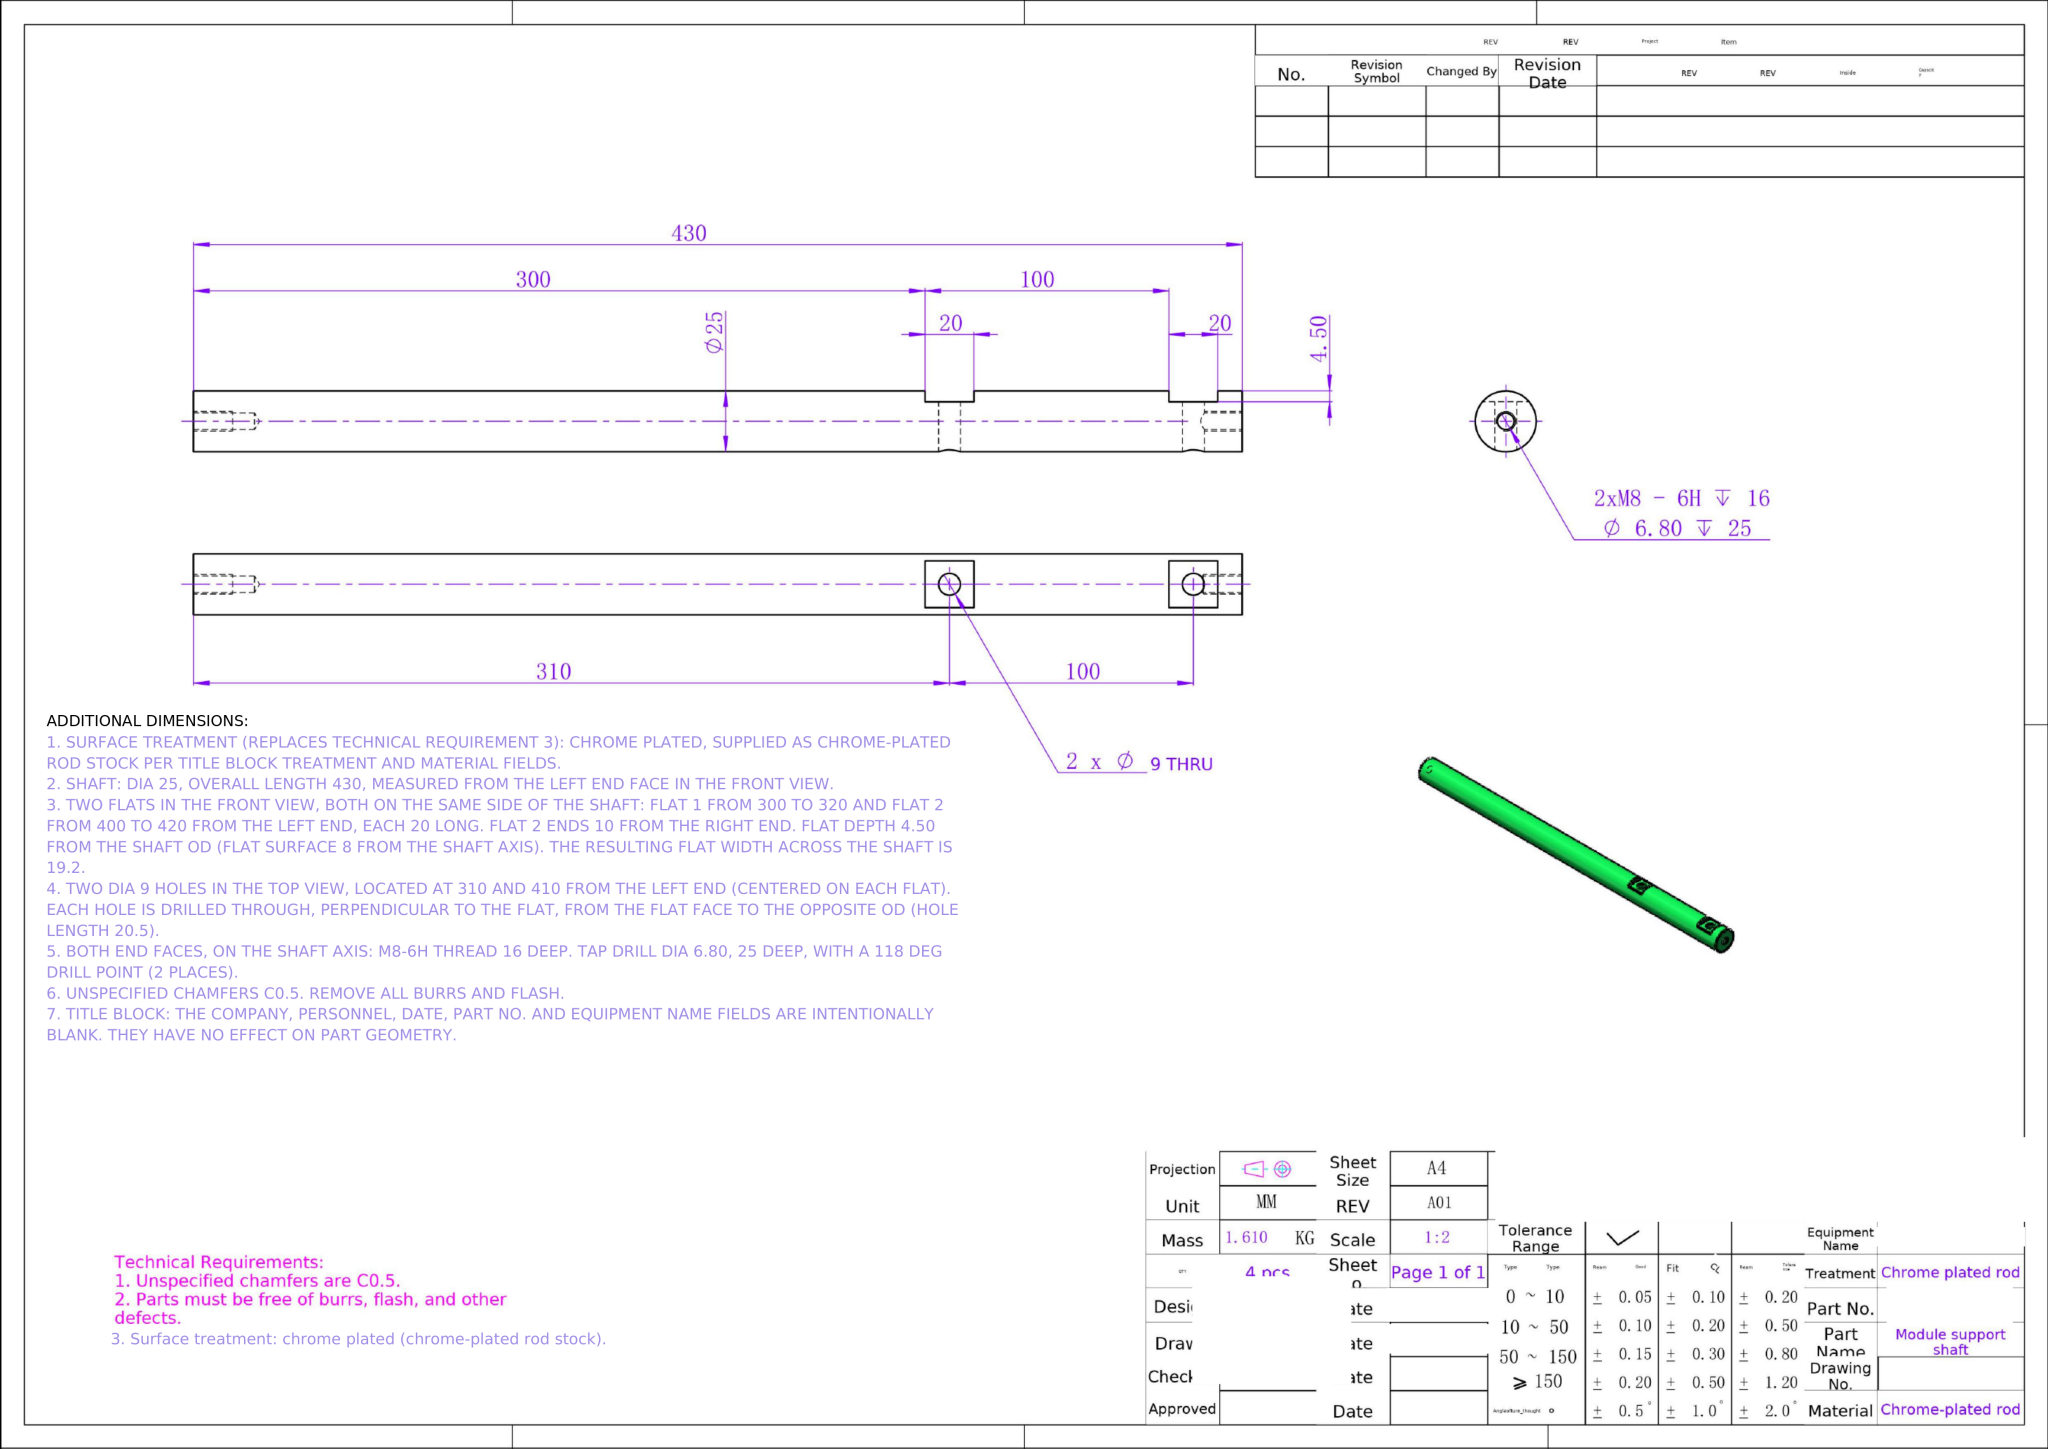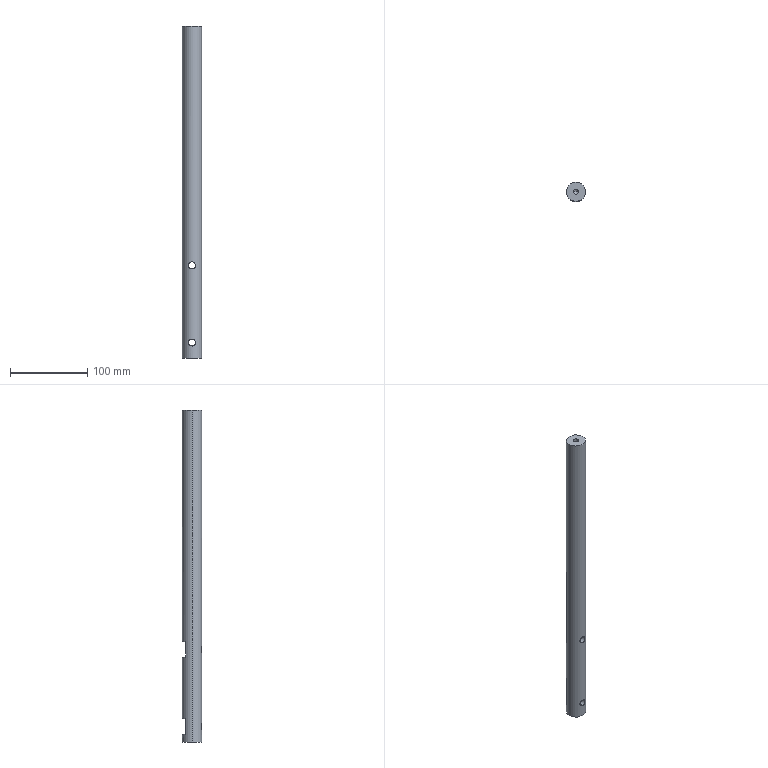Part | NX | mm | Dual-Bore Cylindrical Support Rod | 1 solid | 20 faces | box 25 x 25 x 430 mm | volume 204582 mm3 | cylinder 10 | plane 8 | cone 2 | commonest cylinder face diameters 6.8 x4 9 x4 25 x2
STEP:
#1=CARTESIAN_POINT('',(43.4,-10.,-412.948));
#2=VERTEX_POINT('',#1);
#3=CARTESIAN_POINT('',(40.,-13.4,-414.5));
#4=VERTEX_POINT('',#3);
#5=CARTESIAN_POINT('',(43.4,-10.,-412.948));
#6=CARTESIAN_POINT('',(43.4,-10.117,-412.948));
#7=CARTESIAN_POINT('',(43.394,-10.235,-412.955));
#8=CARTESIAN_POINT('',(43.37,-10.467,-412.982));
#9=CARTESIAN_POINT('',(43.352,-10.581,-413.003));
#10=CARTESIAN_POINT('',(43.282,-10.916,-413.079));
#11=CARTESIAN_POINT('',(43.214,-11.132,-413.152));
#12=CARTESIAN_POINT('',(42.958,-11.733,-413.4));
#13=CARTESIAN_POINT('',(42.716,-12.089,-413.605));
#14=CARTESIAN_POINT('',(42.267,-12.542,-413.891));
#15=CARTESIAN_POINT('',(42.101,-12.682,-413.984));
#16=CARTESIAN_POINT('',(41.742,-12.928,-414.154));
#17=CARTESIAN_POINT('',(41.549,-13.035,-414.23));
#18=CARTESIAN_POINT('',(41.137,-13.212,-414.359));
#19=CARTESIAN_POINT('',(40.916,-13.282,-414.412));
#20=CARTESIAN_POINT('',(40.468,-13.375,-414.481));
#21=CARTESIAN_POINT('',(40.235,-13.4,-414.5));
#22=CARTESIAN_POINT('',(40.,-13.4,-414.5));
#23=B_SPLINE_CURVE_WITH_KNOTS('',3,(#5,#6,#7,#8,#9,#10,#11,#12,#13,#14,#15,#16,#17,#18,#19,#20,#21,#22),.UNSPECIFIED.,.F.,.F.,(4,2,2,2,2,2,2,2,4),(0.01113,0.01148,0.01183,0.01252,0.01391,0.01461,0.0153,0.016,0.01669),.UNSPECIFIED.);
#24=EDGE_CURVE('',#2,#4,#23,.T.);
#25=ORIENTED_EDGE('',*,*,#24,.F.);
#26=CARTESIAN_POINT('',(43.4,-10.,-430.));
#27=VERTEX_POINT('',#26);
#28=CARTESIAN_POINT('',(43.4,-10.,-430.));
#29=DIRECTION('',(0.,0.,-1.));
#30=VECTOR('',#29,1000.);
#31=LINE('',#28,#30);
#32=EDGE_CURVE('',#2,#27,#31,.T.);
#33=ORIENTED_EDGE('',*,*,#32,.T.);
#34=CARTESIAN_POINT('',(36.6,-10.,-430.));
#35=VERTEX_POINT('',#34);
#36=CARTESIAN_POINT('',(40.,-10.,-430.));
#37=DIRECTION('',(0.,0.,-1.));
#38=DIRECTION('',(-1.,0.,0.));
#39=AXIS2_PLACEMENT_3D('',#36,#37,#38);
#40=CIRCLE('',#39,3.4);
#41=EDGE_CURVE('',#27,#35,#40,.T.);
#42=ORIENTED_EDGE('',*,*,#41,.T.);
#43=CARTESIAN_POINT('',(36.6,-10.,-412.948));
#44=VERTEX_POINT('',#43);
#45=CARTESIAN_POINT('',(36.6,-10.,-430.));
#46=DIRECTION('',(0.,0.,-1.));
#47=VECTOR('',#46,1000.);
#48=LINE('',#45,#47);
#49=EDGE_CURVE('',#44,#35,#48,.T.);
#50=ORIENTED_EDGE('',*,*,#49,.F.);
#51=CARTESIAN_POINT('',(40.,-13.4,-414.5));
#52=CARTESIAN_POINT('',(39.765,-13.4,-414.5));
#53=CARTESIAN_POINT('',(39.535,-13.376,-414.482));
#54=CARTESIAN_POINT('',(39.083,-13.282,-414.411));
#55=CARTESIAN_POINT('',(38.862,-13.212,-414.359));
#56=CARTESIAN_POINT('',(38.451,-13.035,-414.231));
#57=CARTESIAN_POINT('',(38.255,-12.926,-414.153));
#58=CARTESIAN_POINT('',(37.897,-12.68,-413.983));
#59=CARTESIAN_POINT('',(37.733,-12.543,-413.891));
#60=CARTESIAN_POINT('',(37.281,-12.086,-413.604));
#61=CARTESIAN_POINT('',(37.044,-11.736,-413.401));
#62=CARTESIAN_POINT('',(36.785,-11.129,-413.151));
#63=CARTESIAN_POINT('',(36.718,-10.918,-413.08));
#64=CARTESIAN_POINT('',(36.625,-10.47,-412.977));
#65=CARTESIAN_POINT('',(36.6,-10.236,-412.948));
#66=CARTESIAN_POINT('',(36.6,-10.,-412.948));
#67=B_SPLINE_CURVE_WITH_KNOTS('',3,(#51,#52,#53,#54,#55,#56,#57,#58,#59,#60,#61,#62,#63,#64,#65,#66),.UNSPECIFIED.,.F.,.F.,(4,2,2,2,2,2,2,4),(0.01669,0.01739,0.01808,0.01878,0.01947,0.02086,0.02155,0.02225),.UNSPECIFIED.);
#68=EDGE_CURVE('',#4,#44,#67,.T.);
#69=ORIENTED_EDGE('',*,*,#68,.F.);
#70=EDGE_LOOP('',(#25,#33,#42,#50,#69));
#71=FACE_OUTER_BOUND('',#70,.T.);
#72=CARTESIAN_POINT('',(40.,-10.,-430.));
#73=DIRECTION('',(0.,0.,-1.));
#74=DIRECTION('',(-1.,0.,0.));
#75=AXIS2_PLACEMENT_3D('',#72,#73,#74);
#76=CYLINDRICAL_SURFACE('',#75,3.4);
#77=ADVANCED_FACE('',(#71),#76,.F.);
#78=CARTESIAN_POINT('',(36.6,-10.,-25.));
#79=VERTEX_POINT('',#78);
#80=CARTESIAN_POINT('',(43.4,-10.,-25.));
#81=VERTEX_POINT('',#80);
#82=CARTESIAN_POINT('',(40.,-10.,-25.));
#83=DIRECTION('',(0.,0.,1.));
#84=DIRECTION('',(1.,0.,0.));
#85=AXIS2_PLACEMENT_3D('',#82,#83,#84);
#86=CIRCLE('',#85,3.4);
#87=EDGE_CURVE('',#79,#81,#86,.T.);
#88=ORIENTED_EDGE('',*,*,#87,.F.);
#89=CARTESIAN_POINT('',(36.6,-10.,0.));
#90=VERTEX_POINT('',#89);
#91=CARTESIAN_POINT('',(36.6,-10.,0.));
#92=DIRECTION('',(0.,0.,1.));
#93=VECTOR('',#92,1000.);
#94=LINE('',#91,#93);
#95=EDGE_CURVE('',#79,#90,#94,.T.);
#96=ORIENTED_EDGE('',*,*,#95,.T.);
#97=CARTESIAN_POINT('',(43.4,-10.,0.));
#98=VERTEX_POINT('',#97);
#99=CARTESIAN_POINT('',(40.,-10.,0.));
#100=DIRECTION('',(0.,0.,1.));
#101=DIRECTION('',(1.,0.,0.));
#102=AXIS2_PLACEMENT_3D('',#99,#100,#101);
#103=CIRCLE('',#102,3.4);
#104=EDGE_CURVE('',#90,#98,#103,.T.);
#105=ORIENTED_EDGE('',*,*,#104,.T.);
#106=CARTESIAN_POINT('',(43.4,-10.,0.));
#107=DIRECTION('',(0.,0.,1.));
#108=VECTOR('',#107,1000.);
#109=LINE('',#106,#108);
#110=EDGE_CURVE('',#81,#98,#109,.T.);
#111=ORIENTED_EDGE('',*,*,#110,.F.);
#112=EDGE_LOOP('',(#88,#96,#105,#111));
#113=FACE_OUTER_BOUND('',#112,.T.);
#114=CARTESIAN_POINT('',(40.,-10.,0.));
#115=DIRECTION('',(0.,0.,1.));
#116=DIRECTION('',(1.,0.,0.));
#117=AXIS2_PLACEMENT_3D('',#114,#115,#116);
#118=CYLINDRICAL_SURFACE('',#117,3.4);
#119=ADVANCED_FACE('',(#113),#118,.F.);
#120=CARTESIAN_POINT('',(40.,-10.,-27.043));
#121=VERTEX_POINT('',#120);
#122=CARTESIAN_POINT('',(43.4,-10.,-25.));
#123=DIRECTION('',(0.8572,0.,0.515));
#124=VECTOR('',#123,1000.);
#125=LINE('',#122,#124);
#126=EDGE_CURVE('',#121,#81,#125,.T.);
#127=ORIENTED_EDGE('',*,*,#126,.F.);
#128=CARTESIAN_POINT('',(36.6,-10.,-25.));
#129=DIRECTION('',(-0.8572,0.,0.515));
#130=VECTOR('',#129,1000.);
#131=LINE('',#128,#130);
#132=EDGE_CURVE('',#121,#79,#131,.T.);
#133=ORIENTED_EDGE('',*,*,#132,.T.);
#134=ORIENTED_EDGE('',*,*,#87,.T.);
#135=EDGE_LOOP('',(#127,#133,#134));
#136=FACE_OUTER_BOUND('',#135,.T.);
#137=CARTESIAN_POINT('',(40.,-10.,-25.));
#138=DIRECTION('',(0.,0.,1.));
#139=DIRECTION('',(1.,0.,0.));
#140=AXIS2_PLACEMENT_3D('',#137,#138,#139);
#141=CONICAL_SURFACE('',#140,3.4,1.03);
#142=ADVANCED_FACE('',(#136),#141,.F.);
#143=CARTESIAN_POINT('',(40.,-22.5,-405.5));
#144=VERTEX_POINT('',#143);
#145=CARTESIAN_POINT('',(40.,-22.5,-414.5));
#146=VERTEX_POINT('',#145);
#147=CARTESIAN_POINT('',(40.,-22.5,-405.5));
#148=CARTESIAN_POINT('',(39.7,-22.5,-405.5));
#149=CARTESIAN_POINT('',(39.405,-22.489,-405.53));
#150=CARTESIAN_POINT('',(38.827,-22.448,-405.646));
#151=CARTESIAN_POINT('',(38.539,-22.417,-405.733));
#152=CARTESIAN_POINT('',(37.995,-22.341,-405.96));
#153=CARTESIAN_POINT('',(37.738,-22.296,-406.099));
#154=CARTESIAN_POINT('',(37.251,-22.196,-406.426));
#155=CARTESIAN_POINT('',(37.022,-22.142,-406.614));
#156=CARTESIAN_POINT('',(36.611,-22.034,-407.025));
#157=CARTESIAN_POINT('',(36.425,-21.979,-407.251));
#158=CARTESIAN_POINT('',(36.097,-21.876,-407.741));
#159=CARTESIAN_POINT('',(35.959,-21.829,-407.999));
#160=CARTESIAN_POINT('',(35.79,-21.77,-408.404));
#161=CARTESIAN_POINT('',(35.74,-21.752,-408.542));
#162=CARTESIAN_POINT('',(35.653,-21.72,-408.825));
#163=CARTESIAN_POINT('',(35.617,-21.706,-408.971));
#164=CARTESIAN_POINT('',(35.529,-21.673,-409.408));
#165=CARTESIAN_POINT('',(35.5,-21.662,-409.701));
#166=CARTESIAN_POINT('',(35.5,-21.662,-410.294));
#167=CARTESIAN_POINT('',(35.53,-21.673,-410.595));
#168=CARTESIAN_POINT('',(35.646,-21.717,-411.174));
#169=CARTESIAN_POINT('',(35.732,-21.749,-411.456));
#170=CARTESIAN_POINT('',(35.96,-21.83,-412.004));
#171=CARTESIAN_POINT('',(36.099,-21.877,-412.263));
#172=CARTESIAN_POINT('',(36.424,-21.979,-412.748));
#173=CARTESIAN_POINT('',(36.613,-22.034,-412.977));
#174=CARTESIAN_POINT('',(37.026,-22.143,-413.39));
#175=CARTESIAN_POINT('',(37.251,-22.196,-413.574));
#176=CARTESIAN_POINT('',(37.737,-22.296,-413.9));
#177=CARTESIAN_POINT('',(38.,-22.342,-414.042));
#178=CARTESIAN_POINT('',(38.541,-22.418,-414.267));
#179=CARTESIAN_POINT('',(38.823,-22.448,-414.353));
#180=CARTESIAN_POINT('',(39.407,-22.489,-414.471));
#181=CARTESIAN_POINT('',(39.704,-22.5,-414.5));
#182=CARTESIAN_POINT('',(40.,-22.5,-414.5));
#183=B_SPLINE_CURVE_WITH_KNOTS('',3,(#147,#148,#149,#150,#151,#152,#153,#154,#155,#156,#157,#158,#159,#160,#161,#162,#163,#164,#165,#166,#167,#168,#169,#170,#171,#172,#173,#174,#175,#176,#177,#178,#179,#180,#181,#182),.UNSPECIFIED.,.F.,.F.,(4,2,2,2,2,2,2,2,2,2,2,2,2,2,2,2,2,4),(0.,0.0008868,0.001774,0.00266,0.003547,0.004434,0.005321,0.005764,0.006208,0.007095,0.007981,0.008868,0.009755,0.01064,0.01153,0.01242,0.0133,0.01419),.UNSPECIFIED.);
#184=EDGE_CURVE('',#144,#146,#183,.T.);
#185=ORIENTED_EDGE('',*,*,#184,.T.);
#186=CARTESIAN_POINT('',(40.,-2.,-414.5));
#187=DIRECTION('',(0.,1.,0.));
#188=VECTOR('',#187,1000.);
#189=LINE('',#186,#188);
#190=EDGE_CURVE('',#146,#4,#189,.T.);
#191=ORIENTED_EDGE('',*,*,#190,.T.);
#192=ORIENTED_EDGE('',*,*,#68,.T.);
#193=CARTESIAN_POINT('',(40.,-6.6,-414.5));
#194=VERTEX_POINT('',#193);
#195=CARTESIAN_POINT('',(36.6,-10.,-412.948));
#196=CARTESIAN_POINT('',(36.6,-9.763,-412.948));
#197=CARTESIAN_POINT('',(36.624,-9.534,-412.977));
#198=CARTESIAN_POINT('',(36.717,-9.088,-413.078));
#199=CARTESIAN_POINT('',(36.785,-8.871,-413.151));
#200=CARTESIAN_POINT('',(37.041,-8.27,-413.398));
#201=CARTESIAN_POINT('',(37.282,-7.913,-413.604));
#202=CARTESIAN_POINT('',(37.731,-7.459,-413.89));
#203=CARTESIAN_POINT('',(37.898,-7.319,-413.984));
#204=CARTESIAN_POINT('',(38.257,-7.073,-414.154));
#205=CARTESIAN_POINT('',(38.449,-6.966,-414.23));
#206=CARTESIAN_POINT('',(38.863,-6.788,-414.359));
#207=CARTESIAN_POINT('',(39.083,-6.718,-414.411));
#208=CARTESIAN_POINT('',(39.532,-6.625,-414.481));
#209=CARTESIAN_POINT('',(39.765,-6.6,-414.5));
#210=CARTESIAN_POINT('',(40.,-6.6,-414.5));
#211=B_SPLINE_CURVE_WITH_KNOTS('',3,(#195,#196,#197,#198,#199,#200,#201,#202,#203,#204,#205,#206,#207,#208,#209,#210),.UNSPECIFIED.,.F.,.F.,(4,2,2,2,2,2,2,4),(0.,0.0006966,0.001393,0.002786,0.003483,0.004179,0.004876,0.005573),.UNSPECIFIED.);
#212=EDGE_CURVE('',#44,#194,#211,.T.);
#213=ORIENTED_EDGE('',*,*,#212,.T.);
#214=CARTESIAN_POINT('',(40.,-2.,-414.5));
#215=VERTEX_POINT('',#214);
#216=CARTESIAN_POINT('',(40.,-2.,-414.5));
#217=DIRECTION('',(0.,1.,0.));
#218=VECTOR('',#217,1000.);
#219=LINE('',#216,#218);
#220=EDGE_CURVE('',#194,#215,#219,.T.);
#221=ORIENTED_EDGE('',*,*,#220,.T.);
#222=CARTESIAN_POINT('',(40.,-2.,-405.5));
#223=VERTEX_POINT('',#222);
#224=CARTESIAN_POINT('',(40.,-2.,-410.));
#225=DIRECTION('',(0.,1.,0.));
#226=DIRECTION('',(0.,0.,1.));
#227=AXIS2_PLACEMENT_3D('',#224,#225,#226);
#228=CIRCLE('',#227,4.5);
#229=EDGE_CURVE('',#215,#223,#228,.T.);
#230=ORIENTED_EDGE('',*,*,#229,.T.);
#231=CARTESIAN_POINT('',(40.,-2.,-405.5));
#232=DIRECTION('',(0.,1.,0.));
#233=VECTOR('',#232,1000.);
#234=LINE('',#231,#233);
#235=EDGE_CURVE('',#144,#223,#234,.T.);
#236=ORIENTED_EDGE('',*,*,#235,.F.);
#237=EDGE_LOOP('',(#185,#191,#192,#213,#221,#230,#236));
#238=FACE_OUTER_BOUND('',#237,.T.);
#239=CARTESIAN_POINT('',(40.,-2.,-410.));
#240=DIRECTION('',(0.,1.,0.));
#241=DIRECTION('',(0.,0.,1.));
#242=AXIS2_PLACEMENT_3D('',#239,#240,#241);
#243=CYLINDRICAL_SURFACE('',#242,4.5);
#244=ADVANCED_FACE('',(#238),#243,.F.);
#245=CARTESIAN_POINT('',(40.,-22.5,-305.5));
#246=VERTEX_POINT('',#245);
#247=CARTESIAN_POINT('',(40.,-22.5,-314.5));
#248=VERTEX_POINT('',#247);
#249=CARTESIAN_POINT('',(40.,-22.5,-305.5));
#250=CARTESIAN_POINT('',(39.7,-22.5,-305.5));
#251=CARTESIAN_POINT('',(39.405,-22.489,-305.53));
#252=CARTESIAN_POINT('',(38.827,-22.448,-305.646));
#253=CARTESIAN_POINT('',(38.539,-22.417,-305.733));
#254=CARTESIAN_POINT('',(37.995,-22.341,-305.96));
#255=CARTESIAN_POINT('',(37.738,-22.296,-306.099));
#256=CARTESIAN_POINT('',(37.251,-22.196,-306.426));
#257=CARTESIAN_POINT('',(37.022,-22.142,-306.614));
#258=CARTESIAN_POINT('',(36.611,-22.034,-307.025));
#259=CARTESIAN_POINT('',(36.425,-21.979,-307.251));
#260=CARTESIAN_POINT('',(36.097,-21.876,-307.741));
#261=CARTESIAN_POINT('',(35.959,-21.829,-307.999));
#262=CARTESIAN_POINT('',(35.79,-21.77,-308.404));
#263=CARTESIAN_POINT('',(35.74,-21.752,-308.542));
#264=CARTESIAN_POINT('',(35.653,-21.72,-308.825));
#265=CARTESIAN_POINT('',(35.617,-21.706,-308.971));
#266=CARTESIAN_POINT('',(35.529,-21.673,-309.408));
#267=CARTESIAN_POINT('',(35.5,-21.662,-309.701));
#268=CARTESIAN_POINT('',(35.5,-21.662,-310.294));
#269=CARTESIAN_POINT('',(35.53,-21.673,-310.595));
#270=CARTESIAN_POINT('',(35.646,-21.717,-311.174));
#271=CARTESIAN_POINT('',(35.732,-21.749,-311.456));
#272=CARTESIAN_POINT('',(35.96,-21.83,-312.004));
#273=CARTESIAN_POINT('',(36.099,-21.877,-312.263));
#274=CARTESIAN_POINT('',(36.424,-21.979,-312.748));
#275=CARTESIAN_POINT('',(36.613,-22.034,-312.977));
#276=CARTESIAN_POINT('',(37.026,-22.143,-313.39));
#277=CARTESIAN_POINT('',(37.251,-22.196,-313.574));
#278=CARTESIAN_POINT('',(37.737,-22.296,-313.9));
#279=CARTESIAN_POINT('',(38.,-22.342,-314.042));
#280=CARTESIAN_POINT('',(38.541,-22.418,-314.267));
#281=CARTESIAN_POINT('',(38.823,-22.448,-314.353));
#282=CARTESIAN_POINT('',(39.407,-22.489,-314.471));
#283=CARTESIAN_POINT('',(39.704,-22.5,-314.5));
#284=CARTESIAN_POINT('',(40.,-22.5,-314.5));
#285=B_SPLINE_CURVE_WITH_KNOTS('',3,(#249,#250,#251,#252,#253,#254,#255,#256,#257,#258,#259,#260,#261,#262,#263,#264,#265,#266,#267,#268,#269,#270,#271,#272,#273,#274,#275,#276,#277,#278,#279,#280,#281,#282,#283,#284),.UNSPECIFIED.,.F.,.F.,(4,2,2,2,2,2,2,2,2,2,2,2,2,2,2,2,2,4),(0.,0.0008868,0.001774,0.00266,0.003547,0.004434,0.005321,0.005764,0.006208,0.007095,0.007981,0.008868,0.009755,0.01064,0.01153,0.01242,0.0133,0.01419),.UNSPECIFIED.);
#286=EDGE_CURVE('',#246,#248,#285,.T.);
#287=ORIENTED_EDGE('',*,*,#286,.T.);
#288=CARTESIAN_POINT('',(40.,-2.,-314.5));
#289=VERTEX_POINT('',#288);
#290=CARTESIAN_POINT('',(40.,-2.,-314.5));
#291=DIRECTION('',(0.,1.,0.));
#292=VECTOR('',#291,1000.);
#293=LINE('',#290,#292);
#294=EDGE_CURVE('',#248,#289,#293,.T.);
#295=ORIENTED_EDGE('',*,*,#294,.T.);
#296=CARTESIAN_POINT('',(40.,-2.,-305.5));
#297=VERTEX_POINT('',#296);
#298=CARTESIAN_POINT('',(40.,-2.,-310.));
#299=DIRECTION('',(0.,1.,0.));
#300=DIRECTION('',(0.,0.,1.));
#301=AXIS2_PLACEMENT_3D('',#298,#299,#300);
#302=CIRCLE('',#301,4.5);
#303=EDGE_CURVE('',#289,#297,#302,.T.);
#304=ORIENTED_EDGE('',*,*,#303,.T.);
#305=CARTESIAN_POINT('',(40.,-2.,-305.5));
#306=DIRECTION('',(0.,1.,0.));
#307=VECTOR('',#306,1000.);
#308=LINE('',#305,#307);
#309=EDGE_CURVE('',#246,#297,#308,.T.);
#310=ORIENTED_EDGE('',*,*,#309,.F.);
#311=EDGE_LOOP('',(#287,#295,#304,#310));
#312=FACE_OUTER_BOUND('',#311,.T.);
#313=CARTESIAN_POINT('',(40.,-2.,-310.));
#314=DIRECTION('',(0.,1.,0.));
#315=DIRECTION('',(0.,0.,1.));
#316=AXIS2_PLACEMENT_3D('',#313,#314,#315);
#317=CYLINDRICAL_SURFACE('',#316,4.5);
#318=ADVANCED_FACE('',(#312),#317,.F.);
#319=CARTESIAN_POINT('',(30.395,-2.,-400.));
#320=VERTEX_POINT('',#319);
#321=CARTESIAN_POINT('',(49.605,-2.,-400.));
#322=VERTEX_POINT('',#321);
#323=CARTESIAN_POINT('',(40.,-10.,-400.));
#324=DIRECTION('',(0.,0.,-1.));
#325=DIRECTION('',(1.,0.,0.));
#326=AXIS2_PLACEMENT_3D('',#323,#324,#325);
#327=CIRCLE('',#326,12.5);
#328=EDGE_CURVE('',#320,#322,#327,.T.);
#329=ORIENTED_EDGE('',*,*,#328,.F.);
#330=CARTESIAN_POINT('',(30.395,-2.,-420.));
#331=VERTEX_POINT('',#330);
#332=CARTESIAN_POINT('',(30.395,-2.,-430.));
#333=DIRECTION('',(0.,0.,1.));
#334=VECTOR('',#333,1000.);
#335=LINE('',#332,#334);
#336=EDGE_CURVE('',#331,#320,#335,.T.);
#337=ORIENTED_EDGE('',*,*,#336,.F.);
#338=CARTESIAN_POINT('',(49.605,-2.,-420.));
#339=VERTEX_POINT('',#338);
#340=CARTESIAN_POINT('',(40.,-10.,-420.));
#341=DIRECTION('',(0.,0.,-1.));
#342=DIRECTION('',(1.,0.,0.));
#343=AXIS2_PLACEMENT_3D('',#340,#341,#342);
#344=CIRCLE('',#343,12.5);
#345=EDGE_CURVE('',#331,#339,#344,.T.);
#346=ORIENTED_EDGE('',*,*,#345,.T.);
#347=CARTESIAN_POINT('',(49.605,-2.,-430.));
#348=DIRECTION('',(0.,0.,-1.));
#349=VECTOR('',#348,1000.);
#350=LINE('',#347,#349);
#351=EDGE_CURVE('',#322,#339,#350,.T.);
#352=ORIENTED_EDGE('',*,*,#351,.F.);
#353=EDGE_LOOP('',(#329,#337,#346,#352));
#354=FACE_BOUND('',#353,.T.);
#355=CARTESIAN_POINT('',(30.395,-2.,-300.));
#356=VERTEX_POINT('',#355);
#357=CARTESIAN_POINT('',(49.605,-2.,-300.));
#358=VERTEX_POINT('',#357);
#359=CARTESIAN_POINT('',(40.,-10.,-300.));
#360=DIRECTION('',(0.,0.,-1.));
#361=DIRECTION('',(1.,0.,0.));
#362=AXIS2_PLACEMENT_3D('',#359,#360,#361);
#363=CIRCLE('',#362,12.5);
#364=EDGE_CURVE('',#356,#358,#363,.T.);
#365=ORIENTED_EDGE('',*,*,#364,.F.);
#366=CARTESIAN_POINT('',(30.395,-2.,-320.));
#367=VERTEX_POINT('',#366);
#368=CARTESIAN_POINT('',(30.395,-2.,-330.));
#369=DIRECTION('',(0.,0.,1.));
#370=VECTOR('',#369,1000.);
#371=LINE('',#368,#370);
#372=EDGE_CURVE('',#367,#356,#371,.T.);
#373=ORIENTED_EDGE('',*,*,#372,.F.);
#374=CARTESIAN_POINT('',(49.605,-2.,-320.));
#375=VERTEX_POINT('',#374);
#376=CARTESIAN_POINT('',(40.,-10.,-320.));
#377=DIRECTION('',(0.,0.,-1.));
#378=DIRECTION('',(1.,0.,0.));
#379=AXIS2_PLACEMENT_3D('',#376,#377,#378);
#380=CIRCLE('',#379,12.5);
#381=EDGE_CURVE('',#367,#375,#380,.T.);
#382=ORIENTED_EDGE('',*,*,#381,.T.);
#383=CARTESIAN_POINT('',(49.605,-2.,-330.));
#384=DIRECTION('',(0.,0.,-1.));
#385=VECTOR('',#384,1000.);
#386=LINE('',#383,#385);
#387=EDGE_CURVE('',#358,#375,#386,.T.);
#388=ORIENTED_EDGE('',*,*,#387,.F.);
#389=EDGE_LOOP('',(#365,#373,#382,#388));
#390=FACE_BOUND('',#389,.T.);
#391=CARTESIAN_POINT('',(52.5,-10.,-430.));
#392=VERTEX_POINT('',#391);
#393=CARTESIAN_POINT('',(27.5,-10.,-430.));
#394=VERTEX_POINT('',#393);
#395=CARTESIAN_POINT('',(40.,-10.,-430.));
#396=DIRECTION('',(0.,0.,1.));
#397=DIRECTION('',(1.,0.,0.));
#398=AXIS2_PLACEMENT_3D('',#395,#396,#397);
#399=CIRCLE('',#398,12.5);
#400=EDGE_CURVE('',#392,#394,#399,.T.);
#401=ORIENTED_EDGE('',*,*,#400,.T.);
#402=CARTESIAN_POINT('',(27.5,-10.,0.));
#403=VERTEX_POINT('',#402);
#404=CARTESIAN_POINT('',(27.5,-10.,-430.));
#405=DIRECTION('',(0.,0.,1.));
#406=VECTOR('',#405,1000.);
#407=LINE('',#404,#406);
#408=EDGE_CURVE('',#394,#403,#407,.T.);
#409=ORIENTED_EDGE('',*,*,#408,.T.);
#410=CARTESIAN_POINT('',(52.5,-10.,0.));
#411=VERTEX_POINT('',#410);
#412=CARTESIAN_POINT('',(40.,-10.,0.));
#413=DIRECTION('',(0.,0.,1.));
#414=DIRECTION('',(1.,0.,0.));
#415=AXIS2_PLACEMENT_3D('',#412,#413,#414);
#416=CIRCLE('',#415,12.5);
#417=EDGE_CURVE('',#411,#403,#416,.T.);
#418=ORIENTED_EDGE('',*,*,#417,.F.);
#419=CARTESIAN_POINT('',(52.5,-10.,-430.));
#420=DIRECTION('',(0.,0.,1.));
#421=VECTOR('',#420,1000.);
#422=LINE('',#419,#421);
#423=EDGE_CURVE('',#392,#411,#422,.T.);
#424=ORIENTED_EDGE('',*,*,#423,.F.);
#425=EDGE_LOOP('',(#401,#409,#418,#424));
#426=FACE_OUTER_BOUND('',#425,.T.);
#427=CARTESIAN_POINT('',(40.,-10.,-430.));
#428=DIRECTION('',(0.,0.,1.));
#429=DIRECTION('',(1.,0.,0.));
#430=AXIS2_PLACEMENT_3D('',#427,#428,#429);
#431=CYLINDRICAL_SURFACE('',#430,12.5);
#432=ADVANCED_FACE('',(#354,#390,#426),#431,.T.);
#433=ORIENTED_EDGE('',*,*,#408,.F.);
#434=CARTESIAN_POINT('',(40.,-10.,-430.));
#435=DIRECTION('',(0.,0.,1.));
#436=DIRECTION('',(1.,0.,0.));
#437=AXIS2_PLACEMENT_3D('',#434,#435,#436);
#438=CIRCLE('',#437,12.5);
#439=EDGE_CURVE('',#394,#392,#438,.T.);
#440=ORIENTED_EDGE('',*,*,#439,.T.);
#441=ORIENTED_EDGE('',*,*,#423,.T.);
#442=CARTESIAN_POINT('',(40.,-10.,0.));
#443=DIRECTION('',(0.,0.,1.));
#444=DIRECTION('',(1.,0.,0.));
#445=AXIS2_PLACEMENT_3D('',#442,#443,#444);
#446=CIRCLE('',#445,12.5);
#447=EDGE_CURVE('',#403,#411,#446,.T.);
#448=ORIENTED_EDGE('',*,*,#447,.F.);
#449=EDGE_LOOP('',(#433,#440,#441,#448));
#450=FACE_OUTER_BOUND('',#449,.T.);
#451=ORIENTED_EDGE('',*,*,#184,.F.);
#452=CARTESIAN_POINT('',(40.,-22.5,-414.5));
#453=CARTESIAN_POINT('',(40.295,-22.5,-414.5));
#454=CARTESIAN_POINT('',(40.594,-22.489,-414.471));
#455=CARTESIAN_POINT('',(41.177,-22.448,-414.353));
#456=CARTESIAN_POINT('',(41.459,-22.418,-414.267));
#457=CARTESIAN_POINT('',(42.002,-22.342,-414.041));
#458=CARTESIAN_POINT('',(42.265,-22.296,-413.899));
#459=CARTESIAN_POINT('',(42.75,-22.196,-413.574));
#460=CARTESIAN_POINT('',(42.976,-22.143,-413.388));
#461=CARTESIAN_POINT('',(43.391,-22.033,-412.972));
#462=CARTESIAN_POINT('',(43.577,-21.978,-412.746));
#463=CARTESIAN_POINT('',(43.901,-21.877,-412.262));
#464=CARTESIAN_POINT('',(44.041,-21.829,-412.001));
#465=CARTESIAN_POINT('',(44.268,-21.749,-411.456));
#466=CARTESIAN_POINT('',(44.354,-21.717,-411.175));
#467=CARTESIAN_POINT('',(44.47,-21.674,-410.596));
#468=CARTESIAN_POINT('',(44.5,-21.662,-410.295));
#469=CARTESIAN_POINT('',(44.5,-21.662,-409.702));
#470=CARTESIAN_POINT('',(44.471,-21.673,-409.408));
#471=CARTESIAN_POINT('',(44.354,-21.717,-408.825));
#472=CARTESIAN_POINT('',(44.266,-21.75,-408.539));
#473=CARTESIAN_POINT('',(44.041,-21.83,-407.998));
#474=CARTESIAN_POINT('',(43.9,-21.877,-407.736));
#475=CARTESIAN_POINT('',(43.573,-21.98,-407.249));
#476=CARTESIAN_POINT('',(43.388,-22.034,-407.024));
#477=CARTESIAN_POINT('',(42.975,-22.143,-406.611));
#478=CARTESIAN_POINT('',(42.746,-22.197,-406.423));
#479=CARTESIAN_POINT('',(42.261,-22.296,-406.098));
#480=CARTESIAN_POINT('',(42.003,-22.342,-405.96));
#481=CARTESIAN_POINT('',(41.594,-22.399,-405.789));
#482=CARTESIAN_POINT('',(41.453,-22.416,-405.739));
#483=CARTESIAN_POINT('',(41.17,-22.446,-405.652));
#484=CARTESIAN_POINT('',(41.027,-22.459,-405.616));
#485=CARTESIAN_POINT('',(40.594,-22.489,-405.53));
#486=CARTESIAN_POINT('',(40.3,-22.5,-405.5));
#487=CARTESIAN_POINT('',(40.,-22.5,-405.5));
#488=B_SPLINE_CURVE_WITH_KNOTS('',3,(#452,#453,#454,#455,#456,#457,#458,#459,#460,#461,#462,#463,#464,#465,#466,#467,#468,#469,#470,#471,#472,#473,#474,#475,#476,#477,#478,#479,#480,#481,#482,#483,#484,#485,#486,#487),.UNSPECIFIED.,.F.,.F.,(4,2,2,2,2,2,2,2,2,2,2,2,2,2,2,2,2,4),(0.01419,0.01508,0.01596,0.01685,0.01774,0.01862,0.01951,0.0204,0.02128,0.02217,0.02306,0.02394,0.02483,0.02572,0.0266,0.02705,0.02749,0.02838),.UNSPECIFIED.);
#489=EDGE_CURVE('',#146,#144,#488,.T.);
#490=ORIENTED_EDGE('',*,*,#489,.F.);
#491=EDGE_LOOP('',(#451,#490));
#492=FACE_BOUND('',#491,.T.);
#493=ORIENTED_EDGE('',*,*,#286,.F.);
#494=CARTESIAN_POINT('',(40.,-22.5,-314.5));
#495=CARTESIAN_POINT('',(40.295,-22.5,-314.5));
#496=CARTESIAN_POINT('',(40.594,-22.489,-314.471));
#497=CARTESIAN_POINT('',(41.177,-22.448,-314.353));
#498=CARTESIAN_POINT('',(41.459,-22.418,-314.267));
#499=CARTESIAN_POINT('',(42.002,-22.342,-314.041));
#500=CARTESIAN_POINT('',(42.265,-22.296,-313.899));
#501=CARTESIAN_POINT('',(42.75,-22.196,-313.574));
#502=CARTESIAN_POINT('',(42.976,-22.143,-313.388));
#503=CARTESIAN_POINT('',(43.391,-22.033,-312.972));
#504=CARTESIAN_POINT('',(43.577,-21.978,-312.746));
#505=CARTESIAN_POINT('',(43.901,-21.877,-312.262));
#506=CARTESIAN_POINT('',(44.041,-21.829,-312.001));
#507=CARTESIAN_POINT('',(44.268,-21.749,-311.456));
#508=CARTESIAN_POINT('',(44.354,-21.717,-311.175));
#509=CARTESIAN_POINT('',(44.47,-21.674,-310.596));
#510=CARTESIAN_POINT('',(44.5,-21.662,-310.295));
#511=CARTESIAN_POINT('',(44.5,-21.662,-309.702));
#512=CARTESIAN_POINT('',(44.471,-21.673,-309.408));
#513=CARTESIAN_POINT('',(44.354,-21.717,-308.825));
#514=CARTESIAN_POINT('',(44.266,-21.75,-308.539));
#515=CARTESIAN_POINT('',(44.041,-21.83,-307.998));
#516=CARTESIAN_POINT('',(43.9,-21.877,-307.736));
#517=CARTESIAN_POINT('',(43.573,-21.98,-307.249));
#518=CARTESIAN_POINT('',(43.388,-22.034,-307.024));
#519=CARTESIAN_POINT('',(42.975,-22.143,-306.611));
#520=CARTESIAN_POINT('',(42.746,-22.197,-306.423));
#521=CARTESIAN_POINT('',(42.261,-22.296,-306.098));
#522=CARTESIAN_POINT('',(42.003,-22.342,-305.96));
#523=CARTESIAN_POINT('',(41.594,-22.399,-305.789));
#524=CARTESIAN_POINT('',(41.453,-22.416,-305.739));
#525=CARTESIAN_POINT('',(41.17,-22.446,-305.652));
#526=CARTESIAN_POINT('',(41.027,-22.459,-305.616));
#527=CARTESIAN_POINT('',(40.594,-22.489,-305.53));
#528=CARTESIAN_POINT('',(40.3,-22.5,-305.5));
#529=CARTESIAN_POINT('',(40.,-22.5,-305.5));
#530=B_SPLINE_CURVE_WITH_KNOTS('',3,(#494,#495,#496,#497,#498,#499,#500,#501,#502,#503,#504,#505,#506,#507,#508,#509,#510,#511,#512,#513,#514,#515,#516,#517,#518,#519,#520,#521,#522,#523,#524,#525,#526,#527,#528,#529),.UNSPECIFIED.,.F.,.F.,(4,2,2,2,2,2,2,2,2,2,2,2,2,2,2,2,2,4),(0.01419,0.01508,0.01596,0.01685,0.01774,0.01862,0.01951,0.0204,0.02128,0.02217,0.02306,0.02394,0.02483,0.02572,0.0266,0.02705,0.02749,0.02838),.UNSPECIFIED.);
#531=EDGE_CURVE('',#248,#246,#530,.T.);
#532=ORIENTED_EDGE('',*,*,#531,.F.);
#533=EDGE_LOOP('',(#493,#532));
#534=FACE_BOUND('',#533,.T.);
#535=CARTESIAN_POINT('',(40.,-10.,-430.));
#536=DIRECTION('',(0.,0.,1.));
#537=DIRECTION('',(1.,0.,0.));
#538=AXIS2_PLACEMENT_3D('',#535,#536,#537);
#539=CYLINDRICAL_SURFACE('',#538,12.5);
#540=ADVANCED_FACE('',(#450,#492,#534),#539,.T.);
#541=CARTESIAN_POINT('',(40.,-10.,-430.));
#542=DIRECTION('',(0.,0.,-1.));
#543=DIRECTION('',(-1.,0.,0.));
#544=AXIS2_PLACEMENT_3D('',#541,#542,#543);
#545=CIRCLE('',#544,3.4);
#546=EDGE_CURVE('',#35,#27,#545,.T.);
#547=ORIENTED_EDGE('',*,*,#546,.F.);
#548=ORIENTED_EDGE('',*,*,#41,.F.);
#549=EDGE_LOOP('',(#547,#548));
#550=FACE_BOUND('',#549,.T.);
#551=ORIENTED_EDGE('',*,*,#400,.F.);
#552=ORIENTED_EDGE('',*,*,#439,.F.);
#553=EDGE_LOOP('',(#551,#552));
#554=FACE_OUTER_BOUND('',#553,.T.);
#555=CARTESIAN_POINT('',(40.,-10.,-430.));
#556=DIRECTION('',(0.,0.,1.));
#557=DIRECTION('',(1.,0.,0.));
#558=AXIS2_PLACEMENT_3D('',#555,#556,#557);
#559=PLANE('',#558);
#560=ADVANCED_FACE('',(#550,#554),#559,.F.);
#561=CARTESIAN_POINT('',(40.,-10.,0.));
#562=DIRECTION('',(0.,0.,1.));
#563=DIRECTION('',(1.,0.,0.));
#564=AXIS2_PLACEMENT_3D('',#561,#562,#563);
#565=CIRCLE('',#564,3.4);
#566=EDGE_CURVE('',#98,#90,#565,.T.);
#567=ORIENTED_EDGE('',*,*,#566,.F.);
#568=ORIENTED_EDGE('',*,*,#104,.F.);
#569=EDGE_LOOP('',(#567,#568));
#570=FACE_BOUND('',#569,.T.);
#571=ORIENTED_EDGE('',*,*,#417,.T.);
#572=ORIENTED_EDGE('',*,*,#447,.T.);
#573=EDGE_LOOP('',(#571,#572));
#574=FACE_OUTER_BOUND('',#573,.T.);
#575=CARTESIAN_POINT('',(40.,-10.,0.));
#576=DIRECTION('',(0.,0.,1.));
#577=DIRECTION('',(1.,0.,0.));
#578=AXIS2_PLACEMENT_3D('',#575,#576,#577);
#579=PLANE('',#578);
#580=ADVANCED_FACE('',(#570,#574),#579,.T.);
#581=CARTESIAN_POINT('',(40.,-2.,-410.));
#582=DIRECTION('',(0.,1.,0.));
#583=DIRECTION('',(0.,0.,1.));
#584=AXIS2_PLACEMENT_3D('',#581,#582,#583);
#585=CIRCLE('',#584,4.5);
#586=EDGE_CURVE('',#223,#215,#585,.T.);
#587=ORIENTED_EDGE('',*,*,#586,.F.);
#588=ORIENTED_EDGE('',*,*,#229,.F.);
#589=EDGE_LOOP('',(#587,#588));
#590=FACE_BOUND('',#589,.T.);
#591=ORIENTED_EDGE('',*,*,#351,.T.);
#592=CARTESIAN_POINT('',(26.051,-2.,-420.));
#593=DIRECTION('',(-1.,0.,0.));
#594=VECTOR('',#593,1000.);
#595=LINE('',#592,#594);
#596=EDGE_CURVE('',#339,#331,#595,.T.);
#597=ORIENTED_EDGE('',*,*,#596,.T.);
#598=ORIENTED_EDGE('',*,*,#336,.T.);
#599=CARTESIAN_POINT('',(26.051,-2.,-400.));
#600=DIRECTION('',(-1.,0.,0.));
#601=VECTOR('',#600,1000.);
#602=LINE('',#599,#601);
#603=EDGE_CURVE('',#322,#320,#602,.T.);
#604=ORIENTED_EDGE('',*,*,#603,.F.);
#605=EDGE_LOOP('',(#591,#597,#598,#604));
#606=FACE_OUTER_BOUND('',#605,.T.);
#607=CARTESIAN_POINT('',(26.051,-2.,-400.));
#608=DIRECTION('',(-0.,-1.,0.));
#609=DIRECTION('',(1.,-0.,0.));
#610=AXIS2_PLACEMENT_3D('',#607,#608,#609);
#611=PLANE('',#610);
#612=ADVANCED_FACE('',(#590,#606),#611,.F.);
#613=ORIENTED_EDGE('',*,*,#328,.T.);
#614=ORIENTED_EDGE('',*,*,#603,.T.);
#615=EDGE_LOOP('',(#613,#614));
#616=FACE_OUTER_BOUND('',#615,.T.);
#617=CARTESIAN_POINT('',(0.,0.,-400.));
#618=DIRECTION('',(0.,0.,1.));
#619=DIRECTION('',(1.,0.,0.));
#620=AXIS2_PLACEMENT_3D('',#617,#618,#619);
#621=PLANE('',#620);
#622=ADVANCED_FACE('',(#616),#621,.F.);
#623=ORIENTED_EDGE('',*,*,#596,.F.);
#624=ORIENTED_EDGE('',*,*,#345,.F.);
#625=EDGE_LOOP('',(#623,#624));
#626=FACE_OUTER_BOUND('',#625,.T.);
#627=CARTESIAN_POINT('',(0.,0.,-420.));
#628=DIRECTION('',(0.,0.,1.));
#629=DIRECTION('',(1.,0.,0.));
#630=AXIS2_PLACEMENT_3D('',#627,#628,#629);
#631=PLANE('',#630);
#632=ADVANCED_FACE('',(#626),#631,.T.);
#633=ORIENTED_EDGE('',*,*,#364,.T.);
#634=CARTESIAN_POINT('',(26.051,-2.,-300.));
#635=DIRECTION('',(-1.,0.,0.));
#636=VECTOR('',#635,1000.);
#637=LINE('',#634,#636);
#638=EDGE_CURVE('',#358,#356,#637,.T.);
#639=ORIENTED_EDGE('',*,*,#638,.T.);
#640=EDGE_LOOP('',(#633,#639));
#641=FACE_OUTER_BOUND('',#640,.T.);
#642=CARTESIAN_POINT('',(0.,0.,-300.));
#643=DIRECTION('',(0.,0.,1.));
#644=DIRECTION('',(1.,0.,0.));
#645=AXIS2_PLACEMENT_3D('',#642,#643,#644);
#646=PLANE('',#645);
#647=ADVANCED_FACE('',(#641),#646,.F.);
#648=CARTESIAN_POINT('',(40.,-2.,-310.));
#649=DIRECTION('',(0.,1.,0.));
#650=DIRECTION('',(0.,0.,1.));
#651=AXIS2_PLACEMENT_3D('',#648,#649,#650);
#652=CIRCLE('',#651,4.5);
#653=EDGE_CURVE('',#297,#289,#652,.T.);
#654=ORIENTED_EDGE('',*,*,#653,.F.);
#655=ORIENTED_EDGE('',*,*,#303,.F.);
#656=EDGE_LOOP('',(#654,#655));
#657=FACE_BOUND('',#656,.T.);
#658=ORIENTED_EDGE('',*,*,#387,.T.);
#659=CARTESIAN_POINT('',(26.051,-2.,-320.));
#660=DIRECTION('',(-1.,0.,0.));
#661=VECTOR('',#660,1000.);
#662=LINE('',#659,#661);
#663=EDGE_CURVE('',#375,#367,#662,.T.);
#664=ORIENTED_EDGE('',*,*,#663,.T.);
#665=ORIENTED_EDGE('',*,*,#372,.T.);
#666=ORIENTED_EDGE('',*,*,#638,.F.);
#667=EDGE_LOOP('',(#658,#664,#665,#666));
#668=FACE_OUTER_BOUND('',#667,.T.);
#669=CARTESIAN_POINT('',(26.051,-2.,-300.));
#670=DIRECTION('',(-0.,-1.,0.));
#671=DIRECTION('',(1.,-0.,0.));
#672=AXIS2_PLACEMENT_3D('',#669,#670,#671);
#673=PLANE('',#672);
#674=ADVANCED_FACE('',(#657,#668),#673,.F.);
#675=ORIENTED_EDGE('',*,*,#663,.F.);
#676=ORIENTED_EDGE('',*,*,#381,.F.);
#677=EDGE_LOOP('',(#675,#676));
#678=FACE_OUTER_BOUND('',#677,.T.);
#679=CARTESIAN_POINT('',(0.,0.,-320.));
#680=DIRECTION('',(0.,0.,1.));
#681=DIRECTION('',(1.,0.,0.));
#682=AXIS2_PLACEMENT_3D('',#679,#680,#681);
#683=PLANE('',#682);
#684=ADVANCED_FACE('',(#678),#683,.T.);
#685=ORIENTED_EDGE('',*,*,#294,.F.);
#686=ORIENTED_EDGE('',*,*,#531,.T.);
#687=ORIENTED_EDGE('',*,*,#309,.T.);
#688=ORIENTED_EDGE('',*,*,#653,.T.);
#689=EDGE_LOOP('',(#685,#686,#687,#688));
#690=FACE_OUTER_BOUND('',#689,.T.);
#691=CARTESIAN_POINT('',(40.,-2.,-310.));
#692=DIRECTION('',(0.,1.,0.));
#693=DIRECTION('',(0.,0.,1.));
#694=AXIS2_PLACEMENT_3D('',#691,#692,#693);
#695=CYLINDRICAL_SURFACE('',#694,4.5);
#696=ADVANCED_FACE('',(#690),#695,.F.);
#697=ORIENTED_EDGE('',*,*,#190,.F.);
#698=ORIENTED_EDGE('',*,*,#489,.T.);
#699=ORIENTED_EDGE('',*,*,#235,.T.);
#700=ORIENTED_EDGE('',*,*,#586,.T.);
#701=ORIENTED_EDGE('',*,*,#220,.F.);
#702=CARTESIAN_POINT('',(40.,-6.6,-414.5));
#703=CARTESIAN_POINT('',(40.235,-6.6,-414.5));
#704=CARTESIAN_POINT('',(40.465,-6.624,-414.482));
#705=CARTESIAN_POINT('',(40.918,-6.718,-414.411));
#706=CARTESIAN_POINT('',(41.138,-6.788,-414.359));
#707=CARTESIAN_POINT('',(41.55,-6.965,-414.23));
#708=CARTESIAN_POINT('',(41.745,-7.074,-414.152));
#709=CARTESIAN_POINT('',(42.104,-7.32,-413.983));
#710=CARTESIAN_POINT('',(42.268,-7.458,-413.891));
#711=CARTESIAN_POINT('',(42.569,-7.763,-413.699));
#712=CARTESIAN_POINT('',(42.704,-7.928,-413.6));
#713=CARTESIAN_POINT('',(42.94,-8.28,-413.41));
#714=CARTESIAN_POINT('',(43.044,-8.469,-413.317));
#715=CARTESIAN_POINT('',(43.215,-8.873,-413.151));
#716=CARTESIAN_POINT('',(43.282,-9.084,-413.079));
#717=CARTESIAN_POINT('',(43.375,-9.533,-412.977));
#718=CARTESIAN_POINT('',(43.4,-9.766,-412.948));
#719=CARTESIAN_POINT('',(43.4,-10.,-412.948));
#720=B_SPLINE_CURVE_WITH_KNOTS('',3,(#702,#703,#704,#705,#706,#707,#708,#709,#710,#711,#712,#713,#714,#715,#716,#717,#718,#719),.UNSPECIFIED.,.F.,.F.,(4,2,2,2,2,2,2,2,4),(0.005573,0.006268,0.006963,0.007658,0.008353,0.009048,0.009743,0.01044,0.01113),.UNSPECIFIED.);
#721=EDGE_CURVE('',#194,#2,#720,.T.);
#722=ORIENTED_EDGE('',*,*,#721,.T.);
#723=ORIENTED_EDGE('',*,*,#24,.T.);
#724=EDGE_LOOP('',(#697,#698,#699,#700,#701,#722,#723));
#725=FACE_OUTER_BOUND('',#724,.T.);
#726=CARTESIAN_POINT('',(40.,-2.,-410.));
#727=DIRECTION('',(0.,1.,0.));
#728=DIRECTION('',(0.,0.,1.));
#729=AXIS2_PLACEMENT_3D('',#726,#727,#728);
#730=CYLINDRICAL_SURFACE('',#729,4.5);
#731=ADVANCED_FACE('',(#725),#730,.F.);
#732=ORIENTED_EDGE('',*,*,#132,.F.);
#733=ORIENTED_EDGE('',*,*,#126,.T.);
#734=CARTESIAN_POINT('',(40.,-10.,-25.));
#735=DIRECTION('',(0.,0.,1.));
#736=DIRECTION('',(1.,0.,0.));
#737=AXIS2_PLACEMENT_3D('',#734,#735,#736);
#738=CIRCLE('',#737,3.4);
#739=EDGE_CURVE('',#81,#79,#738,.T.);
#740=ORIENTED_EDGE('',*,*,#739,.T.);
#741=EDGE_LOOP('',(#732,#733,#740));
#742=FACE_OUTER_BOUND('',#741,.T.);
#743=CARTESIAN_POINT('',(40.,-10.,-25.));
#744=DIRECTION('',(0.,0.,1.));
#745=DIRECTION('',(1.,0.,0.));
#746=AXIS2_PLACEMENT_3D('',#743,#744,#745);
#747=CONICAL_SURFACE('',#746,3.4,1.03);
#748=ADVANCED_FACE('',(#742),#747,.F.);
#749=ORIENTED_EDGE('',*,*,#95,.F.);
#750=ORIENTED_EDGE('',*,*,#739,.F.);
#751=ORIENTED_EDGE('',*,*,#110,.T.);
#752=ORIENTED_EDGE('',*,*,#566,.T.);
#753=EDGE_LOOP('',(#749,#750,#751,#752));
#754=FACE_OUTER_BOUND('',#753,.T.);
#755=CARTESIAN_POINT('',(40.,-10.,0.));
#756=DIRECTION('',(0.,0.,1.));
#757=DIRECTION('',(1.,0.,0.));
#758=AXIS2_PLACEMENT_3D('',#755,#756,#757);
#759=CYLINDRICAL_SURFACE('',#758,3.4);
#760=ADVANCED_FACE('',(#754),#759,.F.);
#761=ORIENTED_EDGE('',*,*,#32,.F.);
#762=ORIENTED_EDGE('',*,*,#721,.F.);
#763=ORIENTED_EDGE('',*,*,#212,.F.);
#764=ORIENTED_EDGE('',*,*,#49,.T.);
#765=ORIENTED_EDGE('',*,*,#546,.T.);
#766=EDGE_LOOP('',(#761,#762,#763,#764,#765));
#767=FACE_OUTER_BOUND('',#766,.T.);
#768=CARTESIAN_POINT('',(40.,-10.,-430.));
#769=DIRECTION('',(0.,0.,-1.));
#770=DIRECTION('',(-1.,0.,0.));
#771=AXIS2_PLACEMENT_3D('',#768,#769,#770);
#772=CYLINDRICAL_SURFACE('',#771,3.4);
#773=ADVANCED_FACE('',(#767),#772,.F.);
#774=CLOSED_SHELL('',(#77,#119,#142,#244,#318,#432,#540,#560,#580,#612,#622,#632,#647,#674,#684,#696,#731,#748,#760,#773));
#775=MANIFOLD_SOLID_BREP('',#774);
#776=CARTESIAN_POINT('',(0.,0.,0.));
#777=DIRECTION('',(0.,0.,1.));
#778=DIRECTION('',(1.,0.,0.));
#779=AXIS2_PLACEMENT_3D('',#776,#777,#778);
#780=(LENGTH_UNIT()NAMED_UNIT(*)SI_UNIT(.MILLI.,.METRE.));
#781=UNCERTAINTY_MEASURE_WITH_UNIT(LENGTH_MEASURE(0.00001),#780,'','');
#782=(NAMED_UNIT(*)PLANE_ANGLE_UNIT()SI_UNIT($,.RADIAN.));
#783=(NAMED_UNIT(*)SI_UNIT($,.STERADIAN.)SOLID_ANGLE_UNIT());
#784=(GEOMETRIC_REPRESENTATION_CONTEXT(3)GLOBAL_UNCERTAINTY_ASSIGNED_CONTEXT((#781))GLOBAL_UNIT_ASSIGNED_CONTEXT((#780,#782,#783))REPRESENTATION_CONTEXT('',''));
#785=ADVANCED_BREP_SHAPE_REPRESENTATION('',(#775,#779),#784);
#786=COLOUR_RGB('',0.7922,0.8196,0.9333);
#787=FILL_AREA_STYLE_COLOUR('',#786);
#788=FILL_AREA_STYLE('',(#787));
#789=SURFACE_STYLE_FILL_AREA(#788);
#790=SURFACE_SIDE_STYLE('',(#789));
#791=SURFACE_STYLE_USAGE(.BOTH.,#790);
#792=PRESENTATION_STYLE_ASSIGNMENT((#791));
#793=STYLED_ITEM('',(#792),#775);
#794=(LENGTH_UNIT()NAMED_UNIT(*)SI_UNIT(.MILLI.,.METRE.));
#795=UNCERTAINTY_MEASURE_WITH_UNIT(LENGTH_MEASURE(0.00001),#794,'','');
#796=(NAMED_UNIT(*)PLANE_ANGLE_UNIT()SI_UNIT($,.RADIAN.));
#797=(NAMED_UNIT(*)SI_UNIT($,.STERADIAN.)SOLID_ANGLE_UNIT());
#798=(GEOMETRIC_REPRESENTATION_CONTEXT(3)GLOBAL_UNCERTAINTY_ASSIGNED_CONTEXT((#795))GLOBAL_UNIT_ASSIGNED_CONTEXT((#794,#796,#797))REPRESENTATION_CONTEXT('',''));
#799=MECHANICAL_DESIGN_GEOMETRIC_PRESENTATION_REPRESENTATION('',(#793),#798);
#800=PRESENTATION_LAYER_ASSIGNMENT('','',(#793));